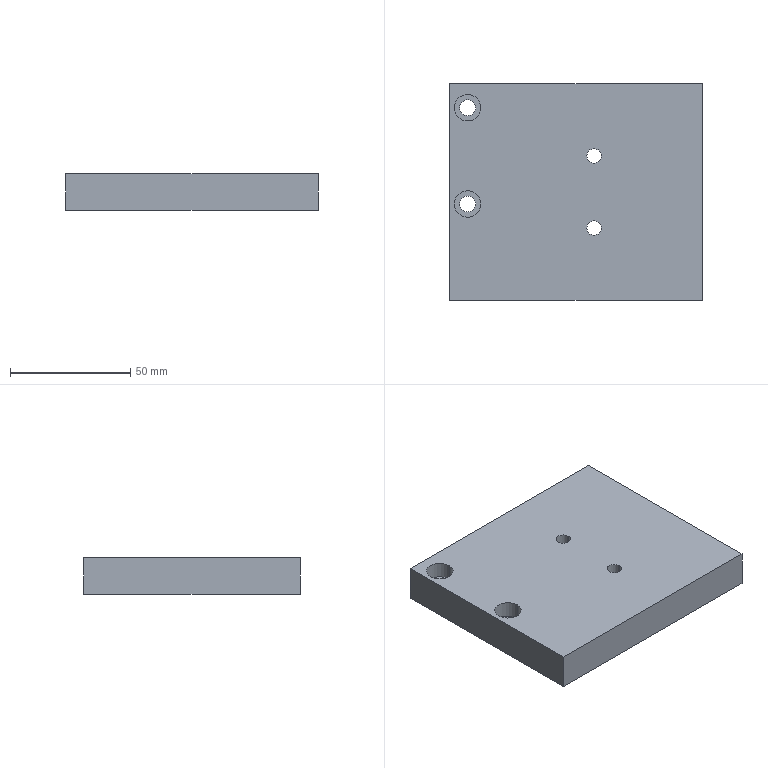Component | SolidWorks | CylinderSupportFrame03-1 | 1 solid | 20 faces | box 105 x 90 x 15 mm | volume 139048 mm3 | cylinder 12 | plane 8 | commonest cylinder face diameters 6 x4 11 x4 6.6 x4
build123d program:
from build123d import *

# Parameters (mm, degrees)
BOSS_EXTRUDE1_DEPTH                               = 60
SKETCH2_W                                         = 105
SKETCH2_H                                         = 15
BOSS_EXTRUDE2_DEPTH                               = 30
HOLE_SIZE_ACCORDING_TO_TYPE_OF_HEX_SO_D           = 6.6
HOLE_SIZE_ACCORDING_TO_TYPE_OF_HEX_SO_DEPTH       = 20
HOLE_SIZE_ACCORDING_TO_TYPE_OF_HEX_SO_CBORE_D     = 11
HOLE_SIZE_ACCORDING_TO_TYPE_OF_HEX_SO_CBORE_DEPTH = 6.8
LPATTERN1_COUNT                                   = 2
LPATTERN1_PITCH                                   = 30
SKETCH5_W                                         = 70
SKETCH5_H                                         = 197
CUT_EXTRUDE1_DEPTH                                = 275.853
HOLE_SIZE_ACCORDING_TO_TYPE_OF_HE_2_D             = 6.6
HOLE_SIZE_ACCORDING_TO_TYPE_OF_HE_2_CBORE_D       = 11
HOLE_SIZE_ACCORDING_TO_TYPE_OF_HE_2_CBORE_DEPTH   = 6.8
M6_TAPPED_HOLE1_D                                 = 6


with BuildPart() as part:
    # Sketch1 → Boss-Extrude1 (new body)
    with BuildSketch(Plane(origin=(0, 0, 0), x_dir=(1, 0, 0), z_dir=(0, 1, 0))):
        Polygon((45, 0), (105, 0), (105, -20), (60, -20), (60, -197), (150, -197), (150, -212), (45, -212), align=None)
    extrude(amount=BOSS_EXTRUDE1_DEPTH)

    # Sketch2 → Boss-Extrude2 (add)
    with BuildSketch(Plane.XZ):
        with Locations((97.5, 204.5)):
            Rectangle(SKETCH2_W, SKETCH2_H)
    extrude(amount=BOSS_EXTRUDE2_DEPTH)

    # Hole Size _ according to_ type of Hex So
    with Locations(Plane(origin=(80, 15, 20), x_dir=(1, 0, 0), z_dir=(0, 0, 1))):
        with Locations((0, 0)):
            hole_size_according_to_type_of_hex_so = CounterBoreHole(HOLE_SIZE_ACCORDING_TO_TYPE_OF_HEX_SO_D / 2, HOLE_SIZE_ACCORDING_TO_TYPE_OF_HEX_SO_CBORE_D / 2, HOLE_SIZE_ACCORDING_TO_TYPE_OF_HEX_SO_CBORE_DEPTH, depth=HOLE_SIZE_ACCORDING_TO_TYPE_OF_HEX_SO_DEPTH)

    # LPattern1: Hole Size _ according to_ type of Hex So ×2
    with Locations(*[(0, i * LPATTERN1_PITCH, 0) for i in range(1, LPATTERN1_COUNT)]):
        add(hole_size_according_to_type_of_hex_so, mode=Mode.SUBTRACT)

    # Sketch5 → Cut-Extrude1 (cut, through all)
    with BuildSketch(Plane(origin=(0, 60, 0), x_dir=(1, 0, 0), z_dir=(0, 1, 0))):
        with Locations((70, -98.5)):
            Rectangle(SKETCH5_W, SKETCH5_H)
    extrude(amount=-CUT_EXTRUDE1_DEPTH, mode=Mode.SUBTRACT)

    # Hole Size _ according to_ type of He 2 (through all)
    with Locations(Plane(origin=(52.5, 50, 212), x_dir=(1, 0, 0), z_dir=(0, 0, 1))):
        with Locations((0, 0), (0, -40)):
            CounterBoreHole(HOLE_SIZE_ACCORDING_TO_TYPE_OF_HE_2_D / 2, HOLE_SIZE_ACCORDING_TO_TYPE_OF_HE_2_CBORE_D / 2, HOLE_SIZE_ACCORDING_TO_TYPE_OF_HE_2_CBORE_DEPTH)

    # M6 Tapped Hole1 (through all)
    with Locations(Plane(origin=(105, 30, 212), x_dir=(1, 0, 0), z_dir=(0, 0, 1))):
        with Locations((0, 0), (0, -30)):
            Hole(M6_TAPPED_HOLE1_D / 2)


solid = part.part

# Placed as in the assembly
solid = solid.moved(Location((-44.66, -15.234, 43.104), (0, 0, 0)))
STEP:
#1=COLOUR_RGB('',0.7922,0.8196,0.9333);
#2=FILL_AREA_STYLE_COLOUR('',#1);
#3=FILL_AREA_STYLE('',(#2));
#4=SURFACE_STYLE_FILL_AREA(#3);
#5=SURFACE_SIDE_STYLE('',(#4));
#6=SURFACE_STYLE_USAGE(.BOTH.,#5);
#7=PRESENTATION_STYLE_ASSIGNMENT((#6));
#8=CARTESIAN_POINT('',(2.257,0.5813,9.453));
#9=VERTEX_POINT('',#8);
#10=CARTESIAN_POINT('',(2.494,0.5813,9.453));
#11=VERTEX_POINT('',#10);
#12=CARTESIAN_POINT('',(2.376,0.5813,9.453));
#13=DIRECTION('',(0.,0.,1.));
#14=DIRECTION('',(1.,0.,0.));
#15=AXIS2_PLACEMENT_3D('',#12,#13,#14);
#16=CIRCLE('',#15,0.1181);
#17=EDGE_CURVE('',#9,#11,#16,.T.);
#18=ORIENTED_EDGE('',*,*,#17,.F.);
#19=CARTESIAN_POINT('',(2.257,0.5813,10.043));
#20=VERTEX_POINT('',#19);
#21=CARTESIAN_POINT('',(2.257,0.5813,10.043));
#22=DIRECTION('',(0.,0.,1.));
#23=VECTOR('',#22,39.37);
#24=LINE('',#21,#23);
#25=EDGE_CURVE('',#9,#20,#24,.T.);
#26=ORIENTED_EDGE('',*,*,#25,.T.);
#27=CARTESIAN_POINT('',(2.494,0.5813,10.043));
#28=VERTEX_POINT('',#27);
#29=CARTESIAN_POINT('',(2.376,0.5813,10.043));
#30=DIRECTION('',(0.,0.,1.));
#31=DIRECTION('',(1.,0.,0.));
#32=AXIS2_PLACEMENT_3D('',#29,#30,#31);
#33=CIRCLE('',#32,0.1181);
#34=EDGE_CURVE('',#20,#28,#33,.T.);
#35=ORIENTED_EDGE('',*,*,#34,.T.);
#36=CARTESIAN_POINT('',(2.494,0.5813,10.043));
#37=DIRECTION('',(0.,0.,1.));
#38=VECTOR('',#37,39.37);
#39=LINE('',#36,#38);
#40=EDGE_CURVE('',#11,#28,#39,.T.);
#41=ORIENTED_EDGE('',*,*,#40,.F.);
#42=EDGE_LOOP('',(#18,#26,#35,#41));
#43=FACE_OUTER_BOUND('',#42,.T.);
#44=CARTESIAN_POINT('',(2.376,0.5813,10.043));
#45=DIRECTION('',(0.,0.,1.));
#46=DIRECTION('',(1.,0.,0.));
#47=AXIS2_PLACEMENT_3D('',#44,#45,#46);
#48=CYLINDRICAL_SURFACE('',#47,0.1181);
#49=ADVANCED_FACE('',(#43),#48,.F.);
#50=CARTESIAN_POINT('',(2.257,-0.5998,9.453));
#51=VERTEX_POINT('',#50);
#52=CARTESIAN_POINT('',(2.494,-0.5998,9.453));
#53=VERTEX_POINT('',#52);
#54=CARTESIAN_POINT('',(2.376,-0.5998,9.453));
#55=DIRECTION('',(0.,0.,1.));
#56=DIRECTION('',(1.,0.,0.));
#57=AXIS2_PLACEMENT_3D('',#54,#55,#56);
#58=CIRCLE('',#57,0.1181);
#59=EDGE_CURVE('',#51,#53,#58,.T.);
#60=ORIENTED_EDGE('',*,*,#59,.F.);
#61=CARTESIAN_POINT('',(2.257,-0.5998,10.043));
#62=VERTEX_POINT('',#61);
#63=CARTESIAN_POINT('',(2.257,-0.5998,10.043));
#64=DIRECTION('',(0.,0.,1.));
#65=VECTOR('',#64,39.37);
#66=LINE('',#63,#65);
#67=EDGE_CURVE('',#51,#62,#66,.T.);
#68=ORIENTED_EDGE('',*,*,#67,.T.);
#69=CARTESIAN_POINT('',(2.494,-0.5998,10.043));
#70=VERTEX_POINT('',#69);
#71=CARTESIAN_POINT('',(2.376,-0.5998,10.043));
#72=DIRECTION('',(0.,0.,1.));
#73=DIRECTION('',(1.,0.,0.));
#74=AXIS2_PLACEMENT_3D('',#71,#72,#73);
#75=CIRCLE('',#74,0.1181);
#76=EDGE_CURVE('',#62,#70,#75,.T.);
#77=ORIENTED_EDGE('',*,*,#76,.T.);
#78=CARTESIAN_POINT('',(2.494,-0.5998,10.043));
#79=DIRECTION('',(0.,0.,1.));
#80=VECTOR('',#79,39.37);
#81=LINE('',#78,#80);
#82=EDGE_CURVE('',#53,#70,#81,.T.);
#83=ORIENTED_EDGE('',*,*,#82,.F.);
#84=EDGE_LOOP('',(#60,#68,#77,#83));
#85=FACE_OUTER_BOUND('',#84,.T.);
#86=CARTESIAN_POINT('',(2.376,-0.5998,10.043));
#87=DIRECTION('',(0.,0.,1.));
#88=DIRECTION('',(1.,0.,0.));
#89=AXIS2_PLACEMENT_3D('',#86,#87,#88);
#90=CYLINDRICAL_SURFACE('',#89,0.1181);
#91=ADVANCED_FACE('',(#85),#90,.F.);
#92=CARTESIAN_POINT('',(0.09214,1.369,9.776));
#93=VERTEX_POINT('',#92);
#94=CARTESIAN_POINT('',(0.5252,1.369,9.776));
#95=VERTEX_POINT('',#94);
#96=CARTESIAN_POINT('',(0.3087,1.369,9.776));
#97=DIRECTION('',(0.,0.,1.));
#98=DIRECTION('',(1.,0.,0.));
#99=AXIS2_PLACEMENT_3D('',#96,#97,#98);
#100=CIRCLE('',#99,0.2165);
#101=EDGE_CURVE('',#93,#95,#100,.T.);
#102=ORIENTED_EDGE('',*,*,#101,.F.);
#103=CARTESIAN_POINT('',(0.09214,1.369,10.043));
#104=VERTEX_POINT('',#103);
#105=CARTESIAN_POINT('',(0.09214,1.369,10.043));
#106=DIRECTION('',(0.,0.,1.));
#107=VECTOR('',#106,39.37);
#108=LINE('',#105,#107);
#109=EDGE_CURVE('',#93,#104,#108,.T.);
#110=ORIENTED_EDGE('',*,*,#109,.T.);
#111=CARTESIAN_POINT('',(0.5252,1.369,10.043));
#112=VERTEX_POINT('',#111);
#113=CARTESIAN_POINT('',(0.3087,1.369,10.043));
#114=DIRECTION('',(0.,0.,1.));
#115=DIRECTION('',(1.,0.,0.));
#116=AXIS2_PLACEMENT_3D('',#113,#114,#115);
#117=CIRCLE('',#116,0.2165);
#118=EDGE_CURVE('',#104,#112,#117,.T.);
#119=ORIENTED_EDGE('',*,*,#118,.T.);
#120=CARTESIAN_POINT('',(0.5252,1.369,10.043));
#121=DIRECTION('',(0.,0.,1.));
#122=VECTOR('',#121,39.37);
#123=LINE('',#120,#122);
#124=EDGE_CURVE('',#95,#112,#123,.T.);
#125=ORIENTED_EDGE('',*,*,#124,.F.);
#126=EDGE_LOOP('',(#102,#110,#119,#125));
#127=FACE_OUTER_BOUND('',#126,.T.);
#128=CARTESIAN_POINT('',(0.3087,1.369,10.043));
#129=DIRECTION('',(0.,0.,1.));
#130=DIRECTION('',(1.,0.,0.));
#131=AXIS2_PLACEMENT_3D('',#128,#129,#130);
#132=CYLINDRICAL_SURFACE('',#131,0.2165);
#133=ADVANCED_FACE('',(#127),#132,.F.);
#134=CARTESIAN_POINT('',(0.1788,1.369,9.453));
#135=VERTEX_POINT('',#134);
#136=CARTESIAN_POINT('',(0.4386,1.369,9.453));
#137=VERTEX_POINT('',#136);
#138=CARTESIAN_POINT('',(0.3087,1.369,9.453));
#139=DIRECTION('',(0.,0.,1.));
#140=DIRECTION('',(1.,0.,0.));
#141=AXIS2_PLACEMENT_3D('',#138,#139,#140);
#142=CIRCLE('',#141,0.1299);
#143=EDGE_CURVE('',#135,#137,#142,.T.);
#144=ORIENTED_EDGE('',*,*,#143,.F.);
#145=CARTESIAN_POINT('',(0.1788,1.369,9.776));
#146=VERTEX_POINT('',#145);
#147=CARTESIAN_POINT('',(0.1788,1.369,10.043));
#148=DIRECTION('',(0.,0.,1.));
#149=VECTOR('',#148,39.37);
#150=LINE('',#147,#149);
#151=EDGE_CURVE('',#135,#146,#150,.T.);
#152=ORIENTED_EDGE('',*,*,#151,.T.);
#153=CARTESIAN_POINT('',(0.4386,1.369,9.776));
#154=VERTEX_POINT('',#153);
#155=CARTESIAN_POINT('',(0.3087,1.369,9.776));
#156=DIRECTION('',(0.,0.,1.));
#157=DIRECTION('',(1.,0.,0.));
#158=AXIS2_PLACEMENT_3D('',#155,#156,#157);
#159=CIRCLE('',#158,0.1299);
#160=EDGE_CURVE('',#146,#154,#159,.T.);
#161=ORIENTED_EDGE('',*,*,#160,.T.);
#162=CARTESIAN_POINT('',(0.4386,1.369,10.043));
#163=DIRECTION('',(0.,0.,1.));
#164=VECTOR('',#163,39.37);
#165=LINE('',#162,#164);
#166=EDGE_CURVE('',#137,#154,#165,.T.);
#167=ORIENTED_EDGE('',*,*,#166,.F.);
#168=EDGE_LOOP('',(#144,#152,#161,#167));
#169=FACE_OUTER_BOUND('',#168,.T.);
#170=CARTESIAN_POINT('',(0.3087,1.369,10.043));
#171=DIRECTION('',(0.,0.,1.));
#172=DIRECTION('',(1.,0.,0.));
#173=AXIS2_PLACEMENT_3D('',#170,#171,#172);
#174=CYLINDRICAL_SURFACE('',#173,0.1299);
#175=ADVANCED_FACE('',(#169),#174,.F.);
#176=CARTESIAN_POINT('',(0.09214,-0.2061,9.776));
#177=VERTEX_POINT('',#176);
#178=CARTESIAN_POINT('',(0.5252,-0.2061,9.776));
#179=VERTEX_POINT('',#178);
#180=CARTESIAN_POINT('',(0.3087,-0.2061,9.776));
#181=DIRECTION('',(0.,0.,1.));
#182=DIRECTION('',(1.,0.,0.));
#183=AXIS2_PLACEMENT_3D('',#180,#181,#182);
#184=CIRCLE('',#183,0.2165);
#185=EDGE_CURVE('',#177,#179,#184,.T.);
#186=ORIENTED_EDGE('',*,*,#185,.F.);
#187=CARTESIAN_POINT('',(0.09214,-0.2061,10.043));
#188=VERTEX_POINT('',#187);
#189=CARTESIAN_POINT('',(0.09214,-0.2061,10.043));
#190=DIRECTION('',(0.,0.,1.));
#191=VECTOR('',#190,39.37);
#192=LINE('',#189,#191);
#193=EDGE_CURVE('',#177,#188,#192,.T.);
#194=ORIENTED_EDGE('',*,*,#193,.T.);
#195=CARTESIAN_POINT('',(0.5252,-0.2061,10.043));
#196=VERTEX_POINT('',#195);
#197=CARTESIAN_POINT('',(0.3087,-0.2061,10.043));
#198=DIRECTION('',(0.,0.,1.));
#199=DIRECTION('',(1.,0.,0.));
#200=AXIS2_PLACEMENT_3D('',#197,#198,#199);
#201=CIRCLE('',#200,0.2165);
#202=EDGE_CURVE('',#188,#196,#201,.T.);
#203=ORIENTED_EDGE('',*,*,#202,.T.);
#204=CARTESIAN_POINT('',(0.5252,-0.2061,10.043));
#205=DIRECTION('',(0.,0.,1.));
#206=VECTOR('',#205,39.37);
#207=LINE('',#204,#206);
#208=EDGE_CURVE('',#179,#196,#207,.T.);
#209=ORIENTED_EDGE('',*,*,#208,.F.);
#210=EDGE_LOOP('',(#186,#194,#203,#209));
#211=FACE_OUTER_BOUND('',#210,.T.);
#212=CARTESIAN_POINT('',(0.3087,-0.2061,10.043));
#213=DIRECTION('',(0.,0.,1.));
#214=DIRECTION('',(1.,0.,0.));
#215=AXIS2_PLACEMENT_3D('',#212,#213,#214);
#216=CYLINDRICAL_SURFACE('',#215,0.2165);
#217=ADVANCED_FACE('',(#211),#216,.F.);
#218=CARTESIAN_POINT('',(0.1788,-0.2061,9.453));
#219=VERTEX_POINT('',#218);
#220=CARTESIAN_POINT('',(0.4386,-0.2061,9.453));
#221=VERTEX_POINT('',#220);
#222=CARTESIAN_POINT('',(0.3087,-0.2061,9.453));
#223=DIRECTION('',(0.,0.,1.));
#224=DIRECTION('',(1.,0.,0.));
#225=AXIS2_PLACEMENT_3D('',#222,#223,#224);
#226=CIRCLE('',#225,0.1299);
#227=EDGE_CURVE('',#219,#221,#226,.T.);
#228=ORIENTED_EDGE('',*,*,#227,.F.);
#229=CARTESIAN_POINT('',(0.1788,-0.2061,9.776));
#230=VERTEX_POINT('',#229);
#231=CARTESIAN_POINT('',(0.1788,-0.2061,10.043));
#232=DIRECTION('',(0.,0.,1.));
#233=VECTOR('',#232,39.37);
#234=LINE('',#231,#233);
#235=EDGE_CURVE('',#219,#230,#234,.T.);
#236=ORIENTED_EDGE('',*,*,#235,.T.);
#237=CARTESIAN_POINT('',(0.4386,-0.2061,9.776));
#238=VERTEX_POINT('',#237);
#239=CARTESIAN_POINT('',(0.3087,-0.2061,9.776));
#240=DIRECTION('',(0.,0.,1.));
#241=DIRECTION('',(1.,0.,0.));
#242=AXIS2_PLACEMENT_3D('',#239,#240,#241);
#243=CIRCLE('',#242,0.1299);
#244=EDGE_CURVE('',#230,#238,#243,.T.);
#245=ORIENTED_EDGE('',*,*,#244,.T.);
#246=CARTESIAN_POINT('',(0.4386,-0.2061,10.043));
#247=DIRECTION('',(0.,0.,1.));
#248=VECTOR('',#247,39.37);
#249=LINE('',#246,#248);
#250=EDGE_CURVE('',#221,#238,#249,.T.);
#251=ORIENTED_EDGE('',*,*,#250,.F.);
#252=EDGE_LOOP('',(#228,#236,#245,#251));
#253=FACE_OUTER_BOUND('',#252,.T.);
#254=CARTESIAN_POINT('',(0.3087,-0.2061,10.043));
#255=DIRECTION('',(0.,0.,1.));
#256=DIRECTION('',(1.,0.,0.));
#257=AXIS2_PLACEMENT_3D('',#254,#255,#256);
#258=CYLINDRICAL_SURFACE('',#257,0.1299);
#259=ADVANCED_FACE('',(#253),#258,.F.);
#260=CARTESIAN_POINT('',(2.376,0.5813,9.453));
#261=DIRECTION('',(0.,0.,1.));
#262=DIRECTION('',(1.,0.,0.));
#263=AXIS2_PLACEMENT_3D('',#260,#261,#262);
#264=CIRCLE('',#263,0.1181);
#265=EDGE_CURVE('',#11,#9,#264,.T.);
#266=ORIENTED_EDGE('',*,*,#265,.T.);
#267=ORIENTED_EDGE('',*,*,#17,.T.);
#268=EDGE_LOOP('',(#266,#267));
#269=FACE_BOUND('',#268,.T.);
#270=CARTESIAN_POINT('',(2.376,-0.5998,9.453));
#271=DIRECTION('',(0.,0.,1.));
#272=DIRECTION('',(1.,0.,0.));
#273=AXIS2_PLACEMENT_3D('',#270,#271,#272);
#274=CIRCLE('',#273,0.1181);
#275=EDGE_CURVE('',#53,#51,#274,.T.);
#276=ORIENTED_EDGE('',*,*,#275,.T.);
#277=ORIENTED_EDGE('',*,*,#59,.T.);
#278=EDGE_LOOP('',(#276,#277));
#279=FACE_BOUND('',#278,.T.);
#280=CARTESIAN_POINT('',(0.3087,1.369,9.453));
#281=DIRECTION('',(0.,0.,1.));
#282=DIRECTION('',(1.,0.,0.));
#283=AXIS2_PLACEMENT_3D('',#280,#281,#282);
#284=CIRCLE('',#283,0.1299);
#285=EDGE_CURVE('',#137,#135,#284,.T.);
#286=ORIENTED_EDGE('',*,*,#285,.T.);
#287=ORIENTED_EDGE('',*,*,#143,.T.);
#288=EDGE_LOOP('',(#286,#287));
#289=FACE_BOUND('',#288,.T.);
#290=CARTESIAN_POINT('',(0.3087,-0.2061,9.453));
#291=DIRECTION('',(0.,0.,1.));
#292=DIRECTION('',(1.,0.,0.));
#293=AXIS2_PLACEMENT_3D('',#290,#291,#292);
#294=CIRCLE('',#293,0.1299);
#295=EDGE_CURVE('',#221,#219,#294,.T.);
#296=ORIENTED_EDGE('',*,*,#295,.T.);
#297=ORIENTED_EDGE('',*,*,#227,.T.);
#298=EDGE_LOOP('',(#296,#297));
#299=FACE_BOUND('',#298,.T.);
#300=CARTESIAN_POINT('',(4.147,1.762,9.453));
#301=VERTEX_POINT('',#300);
#302=CARTESIAN_POINT('',(4.147,-1.781,9.453));
#303=VERTEX_POINT('',#302);
#304=CARTESIAN_POINT('',(4.147,1.762,9.453));
#305=DIRECTION('',(0.,-1.,0.));
#306=VECTOR('',#305,39.37);
#307=LINE('',#304,#306);
#308=EDGE_CURVE('',#301,#303,#307,.T.);
#309=ORIENTED_EDGE('',*,*,#308,.T.);
#310=CARTESIAN_POINT('',(0.0134,-1.781,9.453));
#311=VERTEX_POINT('',#310);
#312=CARTESIAN_POINT('',(4.147,-1.781,9.453));
#313=DIRECTION('',(1.,0.,0.));
#314=VECTOR('',#313,39.37);
#315=LINE('',#312,#314);
#316=EDGE_CURVE('',#311,#303,#315,.T.);
#317=ORIENTED_EDGE('',*,*,#316,.F.);
#318=CARTESIAN_POINT('',(0.0134,1.762,9.453));
#319=VERTEX_POINT('',#318);
#320=CARTESIAN_POINT('',(0.0134,-1.781,9.453));
#321=DIRECTION('',(0.,1.,0.));
#322=VECTOR('',#321,39.37);
#323=LINE('',#320,#322);
#324=EDGE_CURVE('',#311,#319,#323,.T.);
#325=ORIENTED_EDGE('',*,*,#324,.T.);
#326=CARTESIAN_POINT('',(0.604,1.762,9.453));
#327=DIRECTION('',(-1.,0.,0.));
#328=VECTOR('',#327,39.37);
#329=LINE('',#326,#328);
#330=EDGE_CURVE('',#301,#319,#329,.T.);
#331=ORIENTED_EDGE('',*,*,#330,.F.);
#332=EDGE_LOOP('',(#309,#317,#325,#331));
#333=FACE_OUTER_BOUND('',#332,.T.);
#334=CARTESIAN_POINT('',(0.604,1.762,9.453));
#335=DIRECTION('',(0.,0.,1.));
#336=DIRECTION('',(1.,0.,-0.));
#337=AXIS2_PLACEMENT_3D('',#334,#335,#336);
#338=PLANE('',#337);
#339=ADVANCED_FACE('',(#269,#279,#289,#299,#333),#338,.F.);
#340=CARTESIAN_POINT('',(0.0134,1.762,10.043));
#341=VERTEX_POINT('',#340);
#342=CARTESIAN_POINT('',(0.0134,1.762,1.697));
#343=DIRECTION('',(0.,0.,1.));
#344=VECTOR('',#343,39.37);
#345=LINE('',#342,#344);
#346=EDGE_CURVE('',#319,#341,#345,.T.);
#347=ORIENTED_EDGE('',*,*,#346,.F.);
#348=ORIENTED_EDGE('',*,*,#324,.F.);
#349=CARTESIAN_POINT('',(0.0134,-1.781,10.043));
#350=VERTEX_POINT('',#349);
#351=CARTESIAN_POINT('',(0.0134,-1.781,9.453));
#352=DIRECTION('',(0.,0.,-1.));
#353=VECTOR('',#352,39.37);
#354=LINE('',#351,#353);
#355=EDGE_CURVE('',#350,#311,#354,.T.);
#356=ORIENTED_EDGE('',*,*,#355,.F.);
#357=CARTESIAN_POINT('',(0.0134,1.762,10.043));
#358=DIRECTION('',(0.,-1.,0.));
#359=VECTOR('',#358,39.37);
#360=LINE('',#357,#359);
#361=EDGE_CURVE('',#341,#350,#360,.T.);
#362=ORIENTED_EDGE('',*,*,#361,.F.);
#363=EDGE_LOOP('',(#347,#348,#356,#362));
#364=FACE_OUTER_BOUND('',#363,.T.);
#365=CARTESIAN_POINT('',(0.0134,1.762,1.697));
#366=DIRECTION('',(1.,0.,-0.));
#367=DIRECTION('',(-0.,0.,-1.));
#368=AXIS2_PLACEMENT_3D('',#365,#366,#367);
#369=PLANE('',#368);
#370=ADVANCED_FACE('',(#364),#369,.F.);
#371=CARTESIAN_POINT('',(2.376,0.5813,10.043));
#372=DIRECTION('',(0.,0.,1.));
#373=DIRECTION('',(1.,0.,0.));
#374=AXIS2_PLACEMENT_3D('',#371,#372,#373);
#375=CIRCLE('',#374,0.1181);
#376=EDGE_CURVE('',#28,#20,#375,.T.);
#377=ORIENTED_EDGE('',*,*,#376,.F.);
#378=ORIENTED_EDGE('',*,*,#34,.F.);
#379=EDGE_LOOP('',(#377,#378));
#380=FACE_BOUND('',#379,.T.);
#381=CARTESIAN_POINT('',(2.376,-0.5998,10.043));
#382=DIRECTION('',(0.,0.,1.));
#383=DIRECTION('',(1.,0.,0.));
#384=AXIS2_PLACEMENT_3D('',#381,#382,#383);
#385=CIRCLE('',#384,0.1181);
#386=EDGE_CURVE('',#70,#62,#385,.T.);
#387=ORIENTED_EDGE('',*,*,#386,.F.);
#388=ORIENTED_EDGE('',*,*,#76,.F.);
#389=EDGE_LOOP('',(#387,#388));
#390=FACE_BOUND('',#389,.T.);
#391=CARTESIAN_POINT('',(0.3087,1.369,10.043));
#392=DIRECTION('',(0.,0.,1.));
#393=DIRECTION('',(1.,0.,0.));
#394=AXIS2_PLACEMENT_3D('',#391,#392,#393);
#395=CIRCLE('',#394,0.2165);
#396=EDGE_CURVE('',#112,#104,#395,.T.);
#397=ORIENTED_EDGE('',*,*,#396,.F.);
#398=ORIENTED_EDGE('',*,*,#118,.F.);
#399=EDGE_LOOP('',(#397,#398));
#400=FACE_BOUND('',#399,.T.);
#401=CARTESIAN_POINT('',(0.3087,-0.2061,10.043));
#402=DIRECTION('',(0.,0.,1.));
#403=DIRECTION('',(1.,0.,0.));
#404=AXIS2_PLACEMENT_3D('',#401,#402,#403);
#405=CIRCLE('',#404,0.2165);
#406=EDGE_CURVE('',#196,#188,#405,.T.);
#407=ORIENTED_EDGE('',*,*,#406,.F.);
#408=ORIENTED_EDGE('',*,*,#202,.F.);
#409=EDGE_LOOP('',(#407,#408));
#410=FACE_BOUND('',#409,.T.);
#411=ORIENTED_EDGE('',*,*,#361,.T.);
#412=CARTESIAN_POINT('',(4.147,-1.781,10.043));
#413=VERTEX_POINT('',#412);
#414=CARTESIAN_POINT('',(4.147,-1.781,10.043));
#415=DIRECTION('',(-1.,0.,0.));
#416=VECTOR('',#415,39.37);
#417=LINE('',#414,#416);
#418=EDGE_CURVE('',#413,#350,#417,.T.);
#419=ORIENTED_EDGE('',*,*,#418,.F.);
#420=CARTESIAN_POINT('',(4.147,1.762,10.043));
#421=VERTEX_POINT('',#420);
#422=CARTESIAN_POINT('',(4.147,1.762,10.043));
#423=DIRECTION('',(0.,-1.,0.));
#424=VECTOR('',#423,39.37);
#425=LINE('',#422,#424);
#426=EDGE_CURVE('',#421,#413,#425,.T.);
#427=ORIENTED_EDGE('',*,*,#426,.F.);
#428=CARTESIAN_POINT('',(0.0134,1.762,10.043));
#429=DIRECTION('',(1.,0.,0.));
#430=VECTOR('',#429,39.37);
#431=LINE('',#428,#430);
#432=EDGE_CURVE('',#341,#421,#431,.T.);
#433=ORIENTED_EDGE('',*,*,#432,.F.);
#434=EDGE_LOOP('',(#411,#419,#427,#433));
#435=FACE_OUTER_BOUND('',#434,.T.);
#436=CARTESIAN_POINT('',(0.0134,1.762,10.043));
#437=DIRECTION('',(0.,0.,-1.));
#438=DIRECTION('',(-1.,0.,0.));
#439=AXIS2_PLACEMENT_3D('',#436,#437,#438);
#440=PLANE('',#439);
#441=ADVANCED_FACE('',(#380,#390,#400,#410,#435),#440,.F.);
#442=ORIENTED_EDGE('',*,*,#426,.T.);
#443=CARTESIAN_POINT('',(4.147,-1.781,9.453));
#444=DIRECTION('',(0.,0.,1.));
#445=VECTOR('',#444,39.37);
#446=LINE('',#443,#445);
#447=EDGE_CURVE('',#303,#413,#446,.T.);
#448=ORIENTED_EDGE('',*,*,#447,.F.);
#449=ORIENTED_EDGE('',*,*,#308,.F.);
#450=CARTESIAN_POINT('',(4.147,1.762,9.453));
#451=DIRECTION('',(0.,0.,-1.));
#452=VECTOR('',#451,39.37);
#453=LINE('',#450,#452);
#454=EDGE_CURVE('',#421,#301,#453,.T.);
#455=ORIENTED_EDGE('',*,*,#454,.F.);
#456=EDGE_LOOP('',(#442,#448,#449,#455));
#457=FACE_OUTER_BOUND('',#456,.T.);
#458=CARTESIAN_POINT('',(4.147,1.762,9.453));
#459=DIRECTION('',(-1.,0.,0.));
#460=DIRECTION('',(0.,0.,1.));
#461=AXIS2_PLACEMENT_3D('',#458,#459,#460);
#462=PLANE('',#461);
#463=ADVANCED_FACE('',(#457),#462,.F.);
#464=ORIENTED_EDGE('',*,*,#330,.T.);
#465=ORIENTED_EDGE('',*,*,#346,.T.);
#466=ORIENTED_EDGE('',*,*,#432,.T.);
#467=ORIENTED_EDGE('',*,*,#454,.T.);
#468=EDGE_LOOP('',(#464,#465,#466,#467));
#469=FACE_OUTER_BOUND('',#468,.T.);
#470=CARTESIAN_POINT('',(-1.758,1.762,1.697));
#471=DIRECTION('',(0.,-1.,0.));
#472=DIRECTION('',(0.,0.,-1.));
#473=AXIS2_PLACEMENT_3D('',#470,#471,#472);
#474=PLANE('',#473);
#475=ADVANCED_FACE('',(#469),#474,.F.);
#476=ORIENTED_EDGE('',*,*,#447,.T.);
#477=ORIENTED_EDGE('',*,*,#418,.T.);
#478=ORIENTED_EDGE('',*,*,#355,.T.);
#479=ORIENTED_EDGE('',*,*,#316,.T.);
#480=EDGE_LOOP('',(#476,#477,#478,#479));
#481=FACE_OUTER_BOUND('',#480,.T.);
#482=CARTESIAN_POINT('',(-1.758,-1.781,1.697));
#483=DIRECTION('',(0.,-1.,0.));
#484=DIRECTION('',(0.,0.,-1.));
#485=AXIS2_PLACEMENT_3D('',#482,#483,#484);
#486=PLANE('',#485);
#487=ADVANCED_FACE('',(#481),#486,.T.);
#488=ORIENTED_EDGE('',*,*,#235,.F.);
#489=ORIENTED_EDGE('',*,*,#295,.F.);
#490=ORIENTED_EDGE('',*,*,#250,.T.);
#491=CARTESIAN_POINT('',(0.3087,-0.2061,9.776));
#492=DIRECTION('',(0.,0.,1.));
#493=DIRECTION('',(1.,0.,0.));
#494=AXIS2_PLACEMENT_3D('',#491,#492,#493);
#495=CIRCLE('',#494,0.1299);
#496=EDGE_CURVE('',#238,#230,#495,.T.);
#497=ORIENTED_EDGE('',*,*,#496,.T.);
#498=EDGE_LOOP('',(#488,#489,#490,#497));
#499=FACE_OUTER_BOUND('',#498,.T.);
#500=CARTESIAN_POINT('',(0.3087,-0.2061,10.043));
#501=DIRECTION('',(0.,0.,1.));
#502=DIRECTION('',(1.,0.,0.));
#503=AXIS2_PLACEMENT_3D('',#500,#501,#502);
#504=CYLINDRICAL_SURFACE('',#503,0.1299);
#505=ADVANCED_FACE('',(#499),#504,.F.);
#506=ORIENTED_EDGE('',*,*,#496,.F.);
#507=ORIENTED_EDGE('',*,*,#244,.F.);
#508=EDGE_LOOP('',(#506,#507));
#509=FACE_BOUND('',#508,.T.);
#510=CARTESIAN_POINT('',(0.3087,-0.2061,9.776));
#511=DIRECTION('',(0.,0.,1.));
#512=DIRECTION('',(1.,0.,0.));
#513=AXIS2_PLACEMENT_3D('',#510,#511,#512);
#514=CIRCLE('',#513,0.2165);
#515=EDGE_CURVE('',#179,#177,#514,.T.);
#516=ORIENTED_EDGE('',*,*,#515,.T.);
#517=ORIENTED_EDGE('',*,*,#185,.T.);
#518=EDGE_LOOP('',(#516,#517));
#519=FACE_OUTER_BOUND('',#518,.T.);
#520=CARTESIAN_POINT('',(0.4386,-0.2061,9.776));
#521=DIRECTION('',(0.,0.,-1.));
#522=DIRECTION('',(-1.,0.,0.));
#523=AXIS2_PLACEMENT_3D('',#520,#521,#522);
#524=PLANE('',#523);
#525=ADVANCED_FACE('',(#509,#519),#524,.F.);
#526=ORIENTED_EDGE('',*,*,#193,.F.);
#527=ORIENTED_EDGE('',*,*,#515,.F.);
#528=ORIENTED_EDGE('',*,*,#208,.T.);
#529=ORIENTED_EDGE('',*,*,#406,.T.);
#530=EDGE_LOOP('',(#526,#527,#528,#529));
#531=FACE_OUTER_BOUND('',#530,.T.);
#532=CARTESIAN_POINT('',(0.3087,-0.2061,10.043));
#533=DIRECTION('',(0.,0.,1.));
#534=DIRECTION('',(1.,0.,0.));
#535=AXIS2_PLACEMENT_3D('',#532,#533,#534);
#536=CYLINDRICAL_SURFACE('',#535,0.2165);
#537=ADVANCED_FACE('',(#531),#536,.F.);
#538=ORIENTED_EDGE('',*,*,#151,.F.);
#539=ORIENTED_EDGE('',*,*,#285,.F.);
#540=ORIENTED_EDGE('',*,*,#166,.T.);
#541=CARTESIAN_POINT('',(0.3087,1.369,9.776));
#542=DIRECTION('',(0.,0.,1.));
#543=DIRECTION('',(1.,0.,0.));
#544=AXIS2_PLACEMENT_3D('',#541,#542,#543);
#545=CIRCLE('',#544,0.1299);
#546=EDGE_CURVE('',#154,#146,#545,.T.);
#547=ORIENTED_EDGE('',*,*,#546,.T.);
#548=EDGE_LOOP('',(#538,#539,#540,#547));
#549=FACE_OUTER_BOUND('',#548,.T.);
#550=CARTESIAN_POINT('',(0.3087,1.369,10.043));
#551=DIRECTION('',(0.,0.,1.));
#552=DIRECTION('',(1.,0.,0.));
#553=AXIS2_PLACEMENT_3D('',#550,#551,#552);
#554=CYLINDRICAL_SURFACE('',#553,0.1299);
#555=ADVANCED_FACE('',(#549),#554,.F.);
#556=ORIENTED_EDGE('',*,*,#546,.F.);
#557=ORIENTED_EDGE('',*,*,#160,.F.);
#558=EDGE_LOOP('',(#556,#557));
#559=FACE_BOUND('',#558,.T.);
#560=CARTESIAN_POINT('',(0.3087,1.369,9.776));
#561=DIRECTION('',(0.,0.,1.));
#562=DIRECTION('',(1.,0.,0.));
#563=AXIS2_PLACEMENT_3D('',#560,#561,#562);
#564=CIRCLE('',#563,0.2165);
#565=EDGE_CURVE('',#95,#93,#564,.T.);
#566=ORIENTED_EDGE('',*,*,#565,.T.);
#567=ORIENTED_EDGE('',*,*,#101,.T.);
#568=EDGE_LOOP('',(#566,#567));
#569=FACE_OUTER_BOUND('',#568,.T.);
#570=CARTESIAN_POINT('',(0.4386,1.369,9.776));
#571=DIRECTION('',(0.,0.,-1.));
#572=DIRECTION('',(-1.,0.,0.));
#573=AXIS2_PLACEMENT_3D('',#570,#571,#572);
#574=PLANE('',#573);
#575=ADVANCED_FACE('',(#559,#569),#574,.F.);
#576=ORIENTED_EDGE('',*,*,#109,.F.);
#577=ORIENTED_EDGE('',*,*,#565,.F.);
#578=ORIENTED_EDGE('',*,*,#124,.T.);
#579=ORIENTED_EDGE('',*,*,#396,.T.);
#580=EDGE_LOOP('',(#576,#577,#578,#579));
#581=FACE_OUTER_BOUND('',#580,.T.);
#582=CARTESIAN_POINT('',(0.3087,1.369,10.043));
#583=DIRECTION('',(0.,0.,1.));
#584=DIRECTION('',(1.,0.,0.));
#585=AXIS2_PLACEMENT_3D('',#582,#583,#584);
#586=CYLINDRICAL_SURFACE('',#585,0.2165);
#587=ADVANCED_FACE('',(#581),#586,.F.);
#588=ORIENTED_EDGE('',*,*,#67,.F.);
#589=ORIENTED_EDGE('',*,*,#275,.F.);
#590=ORIENTED_EDGE('',*,*,#82,.T.);
#591=ORIENTED_EDGE('',*,*,#386,.T.);
#592=EDGE_LOOP('',(#588,#589,#590,#591));
#593=FACE_OUTER_BOUND('',#592,.T.);
#594=CARTESIAN_POINT('',(2.376,-0.5998,10.043));
#595=DIRECTION('',(0.,0.,1.));
#596=DIRECTION('',(1.,0.,0.));
#597=AXIS2_PLACEMENT_3D('',#594,#595,#596);
#598=CYLINDRICAL_SURFACE('',#597,0.1181);
#599=ADVANCED_FACE('',(#593),#598,.F.);
#600=ORIENTED_EDGE('',*,*,#25,.F.);
#601=ORIENTED_EDGE('',*,*,#265,.F.);
#602=ORIENTED_EDGE('',*,*,#40,.T.);
#603=ORIENTED_EDGE('',*,*,#376,.T.);
#604=EDGE_LOOP('',(#600,#601,#602,#603));
#605=FACE_OUTER_BOUND('',#604,.T.);
#606=CARTESIAN_POINT('',(2.376,0.5813,10.043));
#607=DIRECTION('',(0.,0.,1.));
#608=DIRECTION('',(1.,0.,0.));
#609=AXIS2_PLACEMENT_3D('',#606,#607,#608);
#610=CYLINDRICAL_SURFACE('',#609,0.1181);
#611=ADVANCED_FACE('',(#605),#610,.F.);
#612=CLOSED_SHELL('',(#49,#91,#133,#175,#217,#259,#339,#370,#441,#463,#475,#487,#505,#525,#537,#555,#575,#587,#599,#611));
#613=MANIFOLD_SOLID_BREP('',#612);
#614=STYLED_ITEM('',(#7),#613);
#615=PRESENTATION_LAYER_ASSIGNMENT('','',(#614));
#616=CARTESIAN_POINT('',(0.,0.,0.));
#617=DIRECTION('',(0.,0.,1.));
#618=DIRECTION('',(1.,0.,0.));
#619=AXIS2_PLACEMENT_3D('',#616,#617,#618);
#620=(LENGTH_UNIT()NAMED_UNIT(*)SI_UNIT($,.METRE.));
#621=LENGTH_MEASURE_WITH_UNIT(LENGTH_MEASURE(0.0254),#620);
#622=DIMENSIONAL_EXPONENTS(1.,0.,0.,0.,0.,0.,0.);
#623=(CONVERSION_BASED_UNIT('',#621)LENGTH_UNIT()NAMED_UNIT(#622));
#624=UNCERTAINTY_MEASURE_WITH_UNIT(LENGTH_MEASURE(0.00001),#623,'','');
#625=(NAMED_UNIT(*)PLANE_ANGLE_UNIT()SI_UNIT($,.RADIAN.));
#626=(NAMED_UNIT(*)SI_UNIT($,.STERADIAN.)SOLID_ANGLE_UNIT());
#627=(GEOMETRIC_REPRESENTATION_CONTEXT(3)GLOBAL_UNCERTAINTY_ASSIGNED_CONTEXT((#624))GLOBAL_UNIT_ASSIGNED_CONTEXT((#623,#625,#626))REPRESENTATION_CONTEXT('',''));
#628=ADVANCED_BREP_SHAPE_REPRESENTATION('',(#613,#619),#627);
#629=(LENGTH_UNIT()NAMED_UNIT(*)SI_UNIT($,.METRE.));
#630=LENGTH_MEASURE_WITH_UNIT(LENGTH_MEASURE(0.0254),#629);
#631=DIMENSIONAL_EXPONENTS(1.,0.,0.,0.,0.,0.,0.);
#632=(CONVERSION_BASED_UNIT('',#630)LENGTH_UNIT()NAMED_UNIT(#631));
#633=UNCERTAINTY_MEASURE_WITH_UNIT(LENGTH_MEASURE(0.00001),#632,'','');
#634=(NAMED_UNIT(*)PLANE_ANGLE_UNIT()SI_UNIT($,.RADIAN.));
#635=(NAMED_UNIT(*)SI_UNIT($,.STERADIAN.)SOLID_ANGLE_UNIT());
#636=(GEOMETRIC_REPRESENTATION_CONTEXT(3)GLOBAL_UNCERTAINTY_ASSIGNED_CONTEXT((#633))GLOBAL_UNIT_ASSIGNED_CONTEXT((#632,#634,#635))REPRESENTATION_CONTEXT('',''));
#637=MECHANICAL_DESIGN_GEOMETRIC_PRESENTATION_REPRESENTATION('',(#614),#636);